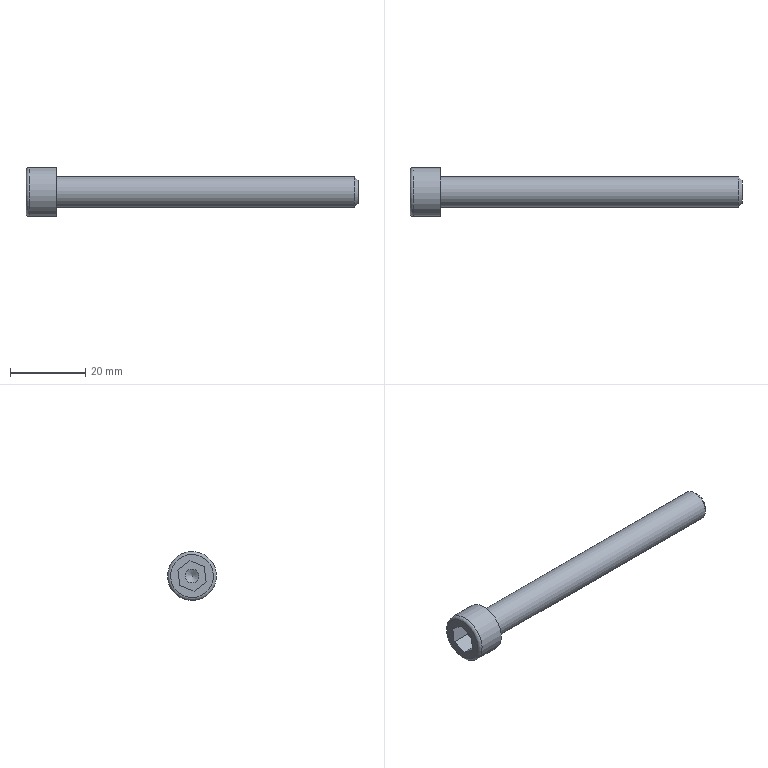Component | NX | GB_T70_1_M8X80_3 | 1 solid | 15 faces | box 88 x 13 x 13 mm | volume 4850 mm3 | plane 10 | cylinder 2 | cone 2 | torus 1 | commonest cylinder face diameters 13 x1 8 x1
STEP:
#1=CARTESIAN_POINT('',(0.,0.,0.));
#2=DIRECTION('',(0.,0.,1.));
#3=DIRECTION('',(1.,0.,0.));
#4=AXIS2_PLACEMENT_3D('',#1,#2,#3);
#5=CARTESIAN_POINT('',(-13.,24.732,-12.177));
#6=VERTEX_POINT('',#5);
#7=CARTESIAN_POINT('',(-13.,30.,-10.));
#8=DIRECTION('',(-1.,0.,0.));
#9=DIRECTION('',(0.,-0.9242,-0.3818));
#10=AXIS2_PLACEMENT_3D('',#7,#8,#9);
#11=CIRCLE('',#10,5.7);
#12=CARTESIAN_POINT('',(-13.,30.,-10.));
#13=DIRECTION('',(1.,0.,0.));
#14=DIRECTION('',(0.,-0.9242,-0.3818));
#15=AXIS2_PLACEMENT_3D('',#12,#13,#14);
#16=PLANE('',#15);
#17=CARTESIAN_POINT('',(5.7,0.));
#18=CARTESIAN_POINT('',(5.7,-9.873));
#19=CARTESIAN_POINT('',(-2.85,-4.936));
#20=CARTESIAN_POINT('',(-11.4,-0.));
#21=CARTESIAN_POINT('',(-2.85,4.936));
#22=CARTESIAN_POINT('',(5.7,9.873));
#23=CARTESIAN_POINT('',(5.7,0.));
#24=(BOUNDED_CURVE()B_SPLINE_CURVE(2,(#17,#18,#19,#20,#21,#22,#23),.UNSPECIFIED.,.T.,.F.)B_SPLINE_CURVE_WITH_KNOTS((1,2,2,2,2,1),(-2.094,0.,2.094,4.189,6.283,8.378),.UNSPECIFIED.)CURVE()GEOMETRIC_REPRESENTATION_ITEM()RATIONAL_B_SPLINE_CURVE((1.,0.5,1.,0.5,1.,0.5,1.))REPRESENTATION_ITEM(''));
#25=(GEOMETRIC_REPRESENTATION_CONTEXT(2)PARAMETRIC_REPRESENTATION_CONTEXT()REPRESENTATION_CONTEXT('',''));
#26=DEFINITIONAL_REPRESENTATION('',(#24),#25);
#27=PCURVE('',#16,#26);
#28=CARTESIAN_POINT('',(-12.2,30.,-10.));
#29=DIRECTION('',(1.,0.,0.));
#30=DIRECTION('',(0.,-0.9242,-0.3818));
#31=AXIS2_PLACEMENT_3D('',#28,#29,#30);
#32=TOROIDAL_SURFACE('',#31,5.7,0.8);
#33=CARTESIAN_POINT('',(6.283,4.712));
#34=DIRECTION('',(-1.,0.));
#35=VECTOR('',#34,1.);
#36=LINE('',#33,#35);
#37=(GEOMETRIC_REPRESENTATION_CONTEXT(2)PARAMETRIC_REPRESENTATION_CONTEXT()REPRESENTATION_CONTEXT('',''));
#38=DEFINITIONAL_REPRESENTATION('',(#36),#37);
#39=PCURVE('',#32,#38);
#40=SURFACE_CURVE('',#11,(#27,#39),.PCURVE_S1.);
#41=EDGE_CURVE('',#6,#6,#40,.T.);
#42=ORIENTED_EDGE('',*,*,#41,.T.);
#43=EDGE_LOOP('',(#42));
#44=FACE_BOUND('',#43,.T.);
#45=CARTESIAN_POINT('',(-13.,26.265,-11.543));
#46=VERTEX_POINT('',#45);
#47=CARTESIAN_POINT('',(-13.,26.796,-7.537));
#48=VERTEX_POINT('',#47);
#49=CARTESIAN_POINT('',(-13.,26.265,-11.543));
#50=DIRECTION('',(0.,0.1314,0.9913));
#51=VECTOR('',#50,1.);
#52=LINE('',#49,#51);
#53=CARTESIAN_POINT('',(4.041,0.));
#54=DIRECTION('',(-0.5,-0.866));
#55=VECTOR('',#54,1.);
#56=LINE('',#53,#55);
#57=(GEOMETRIC_REPRESENTATION_CONTEXT(2)PARAMETRIC_REPRESENTATION_CONTEXT()REPRESENTATION_CONTEXT('',''));
#58=DEFINITIONAL_REPRESENTATION('',(#56),#57);
#59=PCURVE('',#16,#58);
#60=CARTESIAN_POINT('',(-8.,26.265,-11.543));
#61=DIRECTION('',(0.,-0.9913,0.1314));
#62=DIRECTION('',(0.,0.1314,0.9913));
#63=AXIS2_PLACEMENT_3D('',#60,#61,#62);
#64=PLANE('',#63);
#65=CARTESIAN_POINT('',(0.,5.));
#66=DIRECTION('',(1.,0.));
#67=VECTOR('',#66,1.);
#68=LINE('',#65,#67);
#69=(GEOMETRIC_REPRESENTATION_CONTEXT(2)PARAMETRIC_REPRESENTATION_CONTEXT()REPRESENTATION_CONTEXT('',''));
#70=DEFINITIONAL_REPRESENTATION('',(#68),#69);
#71=PCURVE('',#64,#70);
#72=SURFACE_CURVE('',#52,(#59,#71),.PCURVE_S1.);
#73=EDGE_CURVE('',#46,#48,#72,.T.);
#74=ORIENTED_EDGE('',*,*,#73,.F.);
#75=CARTESIAN_POINT('',(-13.,29.469,-14.006));
#76=VERTEX_POINT('',#75);
#77=CARTESIAN_POINT('',(-13.,29.469,-14.006));
#78=DIRECTION('',(0.,-0.7928,0.6095));
#79=VECTOR('',#78,1.);
#80=LINE('',#77,#79);
#81=CARTESIAN_POINT('',(2.021,3.5));
#82=DIRECTION('',(0.5,-0.866));
#83=VECTOR('',#82,1.);
#84=LINE('',#81,#83);
#85=(GEOMETRIC_REPRESENTATION_CONTEXT(2)PARAMETRIC_REPRESENTATION_CONTEXT()REPRESENTATION_CONTEXT('',''));
#86=DEFINITIONAL_REPRESENTATION('',(#84),#85);
#87=PCURVE('',#16,#86);
#88=CARTESIAN_POINT('',(-8.,29.469,-14.006));
#89=DIRECTION('',(0.,-0.6095,-0.7928));
#90=DIRECTION('',(0.,-0.7928,0.6095));
#91=AXIS2_PLACEMENT_3D('',#88,#89,#90);
#92=PLANE('',#91);
#93=CARTESIAN_POINT('',(0.,5.));
#94=DIRECTION('',(1.,0.));
#95=VECTOR('',#94,1.);
#96=LINE('',#93,#95);
#97=(GEOMETRIC_REPRESENTATION_CONTEXT(2)PARAMETRIC_REPRESENTATION_CONTEXT()REPRESENTATION_CONTEXT('',''));
#98=DEFINITIONAL_REPRESENTATION('',(#96),#97);
#99=PCURVE('',#92,#98);
#100=SURFACE_CURVE('',#80,(#87,#99),.PCURVE_S1.);
#101=EDGE_CURVE('',#76,#46,#100,.T.);
#102=ORIENTED_EDGE('',*,*,#101,.F.);
#103=CARTESIAN_POINT('',(-13.,33.204,-12.463));
#104=VERTEX_POINT('',#103);
#105=CARTESIAN_POINT('',(-13.,33.204,-12.463));
#106=DIRECTION('',(0.,-0.9242,-0.3818));
#107=VECTOR('',#106,1.);
#108=LINE('',#105,#107);
#109=CARTESIAN_POINT('',(-2.021,3.5));
#110=DIRECTION('',(1.,0.));
#111=VECTOR('',#110,1.);
#112=LINE('',#109,#111);
#113=(GEOMETRIC_REPRESENTATION_CONTEXT(2)PARAMETRIC_REPRESENTATION_CONTEXT()REPRESENTATION_CONTEXT('',''));
#114=DEFINITIONAL_REPRESENTATION('',(#112),#113);
#115=PCURVE('',#16,#114);
#116=CARTESIAN_POINT('',(-8.,33.204,-12.463));
#117=DIRECTION('',(0.,0.3818,-0.9242));
#118=DIRECTION('',(0.,-0.9242,-0.3818));
#119=AXIS2_PLACEMENT_3D('',#116,#117,#118);
#120=PLANE('',#119);
#121=CARTESIAN_POINT('',(0.,5.));
#122=DIRECTION('',(1.,0.));
#123=VECTOR('',#122,1.);
#124=LINE('',#121,#123);
#125=(GEOMETRIC_REPRESENTATION_CONTEXT(2)PARAMETRIC_REPRESENTATION_CONTEXT()REPRESENTATION_CONTEXT('',''));
#126=DEFINITIONAL_REPRESENTATION('',(#124),#125);
#127=PCURVE('',#120,#126);
#128=SURFACE_CURVE('',#108,(#115,#127),.PCURVE_S1.);
#129=EDGE_CURVE('',#104,#76,#128,.T.);
#130=ORIENTED_EDGE('',*,*,#129,.F.);
#131=CARTESIAN_POINT('',(-13.,33.735,-8.457));
#132=VERTEX_POINT('',#131);
#133=CARTESIAN_POINT('',(-13.,33.735,-8.457));
#134=DIRECTION('',(0.,-0.1314,-0.9913));
#135=VECTOR('',#134,1.);
#136=LINE('',#133,#135);
#137=CARTESIAN_POINT('',(-4.041,-0.));
#138=DIRECTION('',(0.5,0.866));
#139=VECTOR('',#138,1.);
#140=LINE('',#137,#139);
#141=(GEOMETRIC_REPRESENTATION_CONTEXT(2)PARAMETRIC_REPRESENTATION_CONTEXT()REPRESENTATION_CONTEXT('',''));
#142=DEFINITIONAL_REPRESENTATION('',(#140),#141);
#143=PCURVE('',#16,#142);
#144=CARTESIAN_POINT('',(-8.,33.735,-8.457));
#145=DIRECTION('',(0.,0.9913,-0.1314));
#146=DIRECTION('',(0.,-0.1314,-0.9913));
#147=AXIS2_PLACEMENT_3D('',#144,#145,#146);
#148=PLANE('',#147);
#149=CARTESIAN_POINT('',(0.,5.));
#150=DIRECTION('',(1.,0.));
#151=VECTOR('',#150,1.);
#152=LINE('',#149,#151);
#153=(GEOMETRIC_REPRESENTATION_CONTEXT(2)PARAMETRIC_REPRESENTATION_CONTEXT()REPRESENTATION_CONTEXT('',''));
#154=DEFINITIONAL_REPRESENTATION('',(#152),#153);
#155=PCURVE('',#148,#154);
#156=SURFACE_CURVE('',#136,(#143,#155),.PCURVE_S1.);
#157=EDGE_CURVE('',#132,#104,#156,.T.);
#158=ORIENTED_EDGE('',*,*,#157,.F.);
#159=CARTESIAN_POINT('',(-13.,30.531,-5.994));
#160=VERTEX_POINT('',#159);
#161=CARTESIAN_POINT('',(-13.,30.531,-5.994));
#162=DIRECTION('',(0.,0.7928,-0.6095));
#163=VECTOR('',#162,1.);
#164=LINE('',#161,#163);
#165=CARTESIAN_POINT('',(-2.021,-3.5));
#166=DIRECTION('',(-0.5,0.866));
#167=VECTOR('',#166,1.);
#168=LINE('',#165,#167);
#169=(GEOMETRIC_REPRESENTATION_CONTEXT(2)PARAMETRIC_REPRESENTATION_CONTEXT()REPRESENTATION_CONTEXT('',''));
#170=DEFINITIONAL_REPRESENTATION('',(#168),#169);
#171=PCURVE('',#16,#170);
#172=CARTESIAN_POINT('',(-8.,30.531,-5.994));
#173=DIRECTION('',(0.,0.6095,0.7928));
#174=DIRECTION('',(0.,0.7928,-0.6095));
#175=AXIS2_PLACEMENT_3D('',#172,#173,#174);
#176=PLANE('',#175);
#177=CARTESIAN_POINT('',(0.,5.));
#178=DIRECTION('',(1.,0.));
#179=VECTOR('',#178,1.);
#180=LINE('',#177,#179);
#181=(GEOMETRIC_REPRESENTATION_CONTEXT(2)PARAMETRIC_REPRESENTATION_CONTEXT()REPRESENTATION_CONTEXT('',''));
#182=DEFINITIONAL_REPRESENTATION('',(#180),#181);
#183=PCURVE('',#176,#182);
#184=SURFACE_CURVE('',#164,(#171,#183),.PCURVE_S1.);
#185=EDGE_CURVE('',#160,#132,#184,.T.);
#186=ORIENTED_EDGE('',*,*,#185,.F.);
#187=CARTESIAN_POINT('',(-13.,26.796,-7.537));
#188=DIRECTION('',(0.,0.9242,0.3818));
#189=VECTOR('',#188,1.);
#190=LINE('',#187,#189);
#191=CARTESIAN_POINT('',(2.021,-3.5));
#192=DIRECTION('',(-1.,-0.));
#193=VECTOR('',#192,1.);
#194=LINE('',#191,#193);
#195=(GEOMETRIC_REPRESENTATION_CONTEXT(2)PARAMETRIC_REPRESENTATION_CONTEXT()REPRESENTATION_CONTEXT('',''));
#196=DEFINITIONAL_REPRESENTATION('',(#194),#195);
#197=PCURVE('',#16,#196);
#198=CARTESIAN_POINT('',(-8.,26.796,-7.537));
#199=DIRECTION('',(0.,-0.3818,0.9242));
#200=DIRECTION('',(0.,0.9242,0.3818));
#201=AXIS2_PLACEMENT_3D('',#198,#199,#200);
#202=PLANE('',#201);
#203=CARTESIAN_POINT('',(0.,5.));
#204=DIRECTION('',(1.,0.));
#205=VECTOR('',#204,1.);
#206=LINE('',#203,#205);
#207=(GEOMETRIC_REPRESENTATION_CONTEXT(2)PARAMETRIC_REPRESENTATION_CONTEXT()REPRESENTATION_CONTEXT('',''));
#208=DEFINITIONAL_REPRESENTATION('',(#206),#207);
#209=PCURVE('',#202,#208);
#210=SURFACE_CURVE('',#190,(#197,#209),.PCURVE_S1.);
#211=EDGE_CURVE('',#48,#160,#210,.T.);
#212=ORIENTED_EDGE('',*,*,#211,.F.);
#213=EDGE_LOOP('',(#74,#102,#130,#158,#186,#212));
#214=FACE_BOUND('',#213,.T.);
#215=ADVANCED_FACE('',(#44,#214),#16,.F.);
#216=CARTESIAN_POINT('',(-12.2,23.993,-12.482));
#217=VERTEX_POINT('',#216);
#218=CARTESIAN_POINT('',(-12.2,30.,-10.));
#219=DIRECTION('',(1.,0.,0.));
#220=DIRECTION('',(0.,-0.9242,-0.3818));
#221=AXIS2_PLACEMENT_3D('',#218,#219,#220);
#222=CIRCLE('',#221,6.5);
#223=CARTESIAN_POINT('',(75.,30.,-10.));
#224=DIRECTION('',(1.,0.,0.));
#225=DIRECTION('',(0.,-0.9242,-0.3818));
#226=AXIS2_PLACEMENT_3D('',#223,#224,#225);
#227=CYLINDRICAL_SURFACE('',#226,6.5);
#228=CARTESIAN_POINT('',(0.,-87.2));
#229=DIRECTION('',(1.,0.));
#230=VECTOR('',#229,1.);
#231=LINE('',#228,#230);
#232=(GEOMETRIC_REPRESENTATION_CONTEXT(2)PARAMETRIC_REPRESENTATION_CONTEXT()REPRESENTATION_CONTEXT('',''));
#233=DEFINITIONAL_REPRESENTATION('',(#231),#232);
#234=PCURVE('',#227,#233);
#235=CARTESIAN_POINT('',(0.,6.283));
#236=DIRECTION('',(1.,0.));
#237=VECTOR('',#236,1.);
#238=LINE('',#235,#237);
#239=(GEOMETRIC_REPRESENTATION_CONTEXT(2)PARAMETRIC_REPRESENTATION_CONTEXT()REPRESENTATION_CONTEXT('',''));
#240=DEFINITIONAL_REPRESENTATION('',(#238),#239);
#241=PCURVE('',#32,#240);
#242=SURFACE_CURVE('',#222,(#234,#241),.PCURVE_S1.);
#243=EDGE_CURVE('',#217,#217,#242,.T.);
#244=ORIENTED_EDGE('',*,*,#243,.T.);
#245=CARTESIAN_POINT('',(-5.,23.993,-12.482));
#246=VERTEX_POINT('',#245);
#247=CARTESIAN_POINT('',(-12.2,23.993,-12.482));
#248=CARTESIAN_POINT('',(-5.,23.993,-12.482));
#249=B_SPLINE_CURVE_WITH_KNOTS('',1,(#247,#248),.UNSPECIFIED.,.F.,.F.,(2,2),(-87.2,-80.),.PIECEWISE_BEZIER_KNOTS.);
#250=CARTESIAN_POINT('',(6.283,0.));
#251=DIRECTION('',(0.,1.));
#252=VECTOR('',#251,1.);
#253=LINE('',#250,#252);
#254=(GEOMETRIC_REPRESENTATION_CONTEXT(2)PARAMETRIC_REPRESENTATION_CONTEXT()REPRESENTATION_CONTEXT('',''));
#255=DEFINITIONAL_REPRESENTATION('',(#253),#254);
#256=PCURVE('',#227,#255);
#257=CARTESIAN_POINT('',(0.,0.));
#258=DIRECTION('',(0.,1.));
#259=VECTOR('',#258,1.);
#260=LINE('',#257,#259);
#261=(GEOMETRIC_REPRESENTATION_CONTEXT(2)PARAMETRIC_REPRESENTATION_CONTEXT()REPRESENTATION_CONTEXT('',''));
#262=DEFINITIONAL_REPRESENTATION('',(#260),#261);
#263=PCURVE('',#227,#262);
#264=SEAM_CURVE('',#249,(#256,#263),.PCURVE_S1.);
#265=EDGE_CURVE('',#217,#246,#264,.T.);
#266=ORIENTED_EDGE('',*,*,#265,.T.);
#267=CARTESIAN_POINT('',(-5.,30.,-10.));
#268=DIRECTION('',(1.,0.,0.));
#269=DIRECTION('',(0.,-0.9242,-0.3818));
#270=AXIS2_PLACEMENT_3D('',#267,#268,#269);
#271=CIRCLE('',#270,6.5);
#272=CARTESIAN_POINT('',(0.,-80.));
#273=DIRECTION('',(1.,0.));
#274=VECTOR('',#273,1.);
#275=LINE('',#272,#274);
#276=(GEOMETRIC_REPRESENTATION_CONTEXT(2)PARAMETRIC_REPRESENTATION_CONTEXT()REPRESENTATION_CONTEXT('',''));
#277=DEFINITIONAL_REPRESENTATION('',(#275),#276);
#278=PCURVE('',#227,#277);
#279=CARTESIAN_POINT('',(-5.,27.518,-3.993));
#280=DIRECTION('',(-1.,0.,0.));
#281=DIRECTION('',(0.,0.9242,0.3818));
#282=AXIS2_PLACEMENT_3D('',#279,#280,#281);
#283=PLANE('',#282);
#284=CARTESIAN_POINT('',(-6.5,6.5));
#285=CARTESIAN_POINT('',(-6.5,17.758));
#286=CARTESIAN_POINT('',(3.25,12.129));
#287=CARTESIAN_POINT('',(13.,6.5));
#288=CARTESIAN_POINT('',(3.25,0.8708));
#289=CARTESIAN_POINT('',(-6.5,-4.758));
#290=CARTESIAN_POINT('',(-6.5,6.5));
#291=(BOUNDED_CURVE()B_SPLINE_CURVE(2,(#284,#285,#286,#287,#288,#289,#290),.UNSPECIFIED.,.T.,.F.)B_SPLINE_CURVE_WITH_KNOTS((1,2,2,2,2,1),(-2.094,0.,2.094,4.189,6.283,8.378),.UNSPECIFIED.)CURVE()GEOMETRIC_REPRESENTATION_ITEM()RATIONAL_B_SPLINE_CURVE((1.,0.5,1.,0.5,1.,0.5,1.))REPRESENTATION_ITEM(''));
#292=(GEOMETRIC_REPRESENTATION_CONTEXT(2)PARAMETRIC_REPRESENTATION_CONTEXT()REPRESENTATION_CONTEXT('',''));
#293=DEFINITIONAL_REPRESENTATION('',(#291),#292);
#294=PCURVE('',#283,#293);
#295=SURFACE_CURVE('',#271,(#278,#294),.PCURVE_S1.);
#296=EDGE_CURVE('',#246,#246,#295,.T.);
#297=ORIENTED_EDGE('',*,*,#296,.F.);
#298=ORIENTED_EDGE('',*,*,#265,.F.);
#299=EDGE_LOOP('',(#244,#266,#297,#298));
#300=FACE_BOUND('',#299,.T.);
#301=ADVANCED_FACE('',(#300),#227,.T.);
#302=CARTESIAN_POINT('',(-5.,26.303,-11.527));
#303=VERTEX_POINT('',#302);
#304=CARTESIAN_POINT('',(-5.,30.,-10.));
#305=DIRECTION('',(1.,0.,0.));
#306=DIRECTION('',(0.,-0.9242,-0.3818));
#307=AXIS2_PLACEMENT_3D('',#304,#305,#306);
#308=CIRCLE('',#307,4.);
#309=CARTESIAN_POINT('',(-4.,6.5));
#310=CARTESIAN_POINT('',(-4.,13.428));
#311=CARTESIAN_POINT('',(2.,9.964));
#312=CARTESIAN_POINT('',(8.,6.5));
#313=CARTESIAN_POINT('',(2.,3.036));
#314=CARTESIAN_POINT('',(-4.,-0.4282));
#315=CARTESIAN_POINT('',(-4.,6.5));
#316=(BOUNDED_CURVE()B_SPLINE_CURVE(2,(#309,#310,#311,#312,#313,#314,#315),.UNSPECIFIED.,.T.,.F.)B_SPLINE_CURVE_WITH_KNOTS((1,2,2,2,2,1),(-2.094,0.,2.094,4.189,6.283,8.378),.UNSPECIFIED.)CURVE()GEOMETRIC_REPRESENTATION_ITEM()RATIONAL_B_SPLINE_CURVE((1.,0.5,1.,0.5,1.,0.5,1.))REPRESENTATION_ITEM(''));
#317=(GEOMETRIC_REPRESENTATION_CONTEXT(2)PARAMETRIC_REPRESENTATION_CONTEXT()REPRESENTATION_CONTEXT('',''));
#318=DEFINITIONAL_REPRESENTATION('',(#316),#317);
#319=PCURVE('',#283,#318);
#320=CARTESIAN_POINT('',(75.,30.,-10.));
#321=DIRECTION('',(1.,0.,0.));
#322=DIRECTION('',(0.,-0.9242,-0.3818));
#323=AXIS2_PLACEMENT_3D('',#320,#321,#322);
#324=CYLINDRICAL_SURFACE('',#323,4.);
#325=CARTESIAN_POINT('',(0.,-80.));
#326=DIRECTION('',(1.,0.));
#327=VECTOR('',#326,1.);
#328=LINE('',#325,#327);
#329=(GEOMETRIC_REPRESENTATION_CONTEXT(2)PARAMETRIC_REPRESENTATION_CONTEXT()REPRESENTATION_CONTEXT('',''));
#330=DEFINITIONAL_REPRESENTATION('',(#328),#329);
#331=PCURVE('',#324,#330);
#332=SURFACE_CURVE('',#308,(#319,#331),.PCURVE_S1.);
#333=EDGE_CURVE('',#303,#303,#332,.T.);
#334=ORIENTED_EDGE('',*,*,#333,.F.);
#335=EDGE_LOOP('',(#334));
#336=FACE_BOUND('',#335,.T.);
#337=ORIENTED_EDGE('',*,*,#296,.T.);
#338=EDGE_LOOP('',(#337));
#339=FACE_BOUND('',#338,.T.);
#340=ADVANCED_FACE('',(#336,#339),#283,.F.);
#341=CARTESIAN_POINT('',(74.,33.697,-8.473));
#342=VERTEX_POINT('',#341);
#343=CARTESIAN_POINT('',(74.,26.303,-11.527));
#344=VERTEX_POINT('',#343);
#345=CARTESIAN_POINT('',(74.,30.,-10.));
#346=DIRECTION('',(-1.,0.,0.));
#347=DIRECTION('',(0.,0.9242,0.3818));
#348=AXIS2_PLACEMENT_3D('',#345,#346,#347);
#349=CIRCLE('',#348,4.);
#350=CARTESIAN_POINT('',(3.142,-1.));
#351=DIRECTION('',(-1.,0.));
#352=VECTOR('',#351,1.);
#353=LINE('',#350,#352);
#354=(GEOMETRIC_REPRESENTATION_CONTEXT(2)PARAMETRIC_REPRESENTATION_CONTEXT()REPRESENTATION_CONTEXT('',''));
#355=DEFINITIONAL_REPRESENTATION('',(#353),#354);
#356=PCURVE('',#324,#355);
#357=CARTESIAN_POINT('',(75.,30.,-10.));
#358=DIRECTION('',(-1.,0.,0.));
#359=DIRECTION('',(0.,0.9242,0.3818));
#360=AXIS2_PLACEMENT_3D('',#357,#358,#359);
#361=CONICAL_SURFACE('',#360,3.,0.7854);
#362=CARTESIAN_POINT('',(0.,1.));
#363=DIRECTION('',(1.,0.));
#364=VECTOR('',#363,1.);
#365=LINE('',#362,#364);
#366=(GEOMETRIC_REPRESENTATION_CONTEXT(2)PARAMETRIC_REPRESENTATION_CONTEXT()REPRESENTATION_CONTEXT('',''));
#367=DEFINITIONAL_REPRESENTATION('',(#365),#366);
#368=PCURVE('',#361,#367);
#369=SURFACE_CURVE('',#349,(#356,#368),.PCURVE_S1.);
#370=EDGE_CURVE('',#342,#344,#369,.T.);
#371=ORIENTED_EDGE('',*,*,#370,.T.);
#372=CARTESIAN_POINT('',(-5.,26.303,-11.527));
#373=CARTESIAN_POINT('',(74.,26.303,-11.527));
#374=B_SPLINE_CURVE_WITH_KNOTS('',1,(#372,#373),.UNSPECIFIED.,.F.,.F.,(2,2),(-80.,-1.),.PIECEWISE_BEZIER_KNOTS.);
#375=CARTESIAN_POINT('',(0.,0.));
#376=DIRECTION('',(0.,1.));
#377=VECTOR('',#376,1.);
#378=LINE('',#375,#377);
#379=(GEOMETRIC_REPRESENTATION_CONTEXT(2)PARAMETRIC_REPRESENTATION_CONTEXT()REPRESENTATION_CONTEXT('',''));
#380=DEFINITIONAL_REPRESENTATION('',(#378),#379);
#381=PCURVE('',#324,#380);
#382=CARTESIAN_POINT('',(6.283,0.));
#383=DIRECTION('',(0.,1.));
#384=VECTOR('',#383,1.);
#385=LINE('',#382,#384);
#386=(GEOMETRIC_REPRESENTATION_CONTEXT(2)PARAMETRIC_REPRESENTATION_CONTEXT()REPRESENTATION_CONTEXT('',''));
#387=DEFINITIONAL_REPRESENTATION('',(#385),#386);
#388=PCURVE('',#324,#387);
#389=SEAM_CURVE('',#374,(#381,#388),.PCURVE_S1.);
#390=EDGE_CURVE('',#303,#344,#389,.T.);
#391=ORIENTED_EDGE('',*,*,#390,.F.);
#392=ORIENTED_EDGE('',*,*,#333,.T.);
#393=ORIENTED_EDGE('',*,*,#390,.T.);
#394=CARTESIAN_POINT('',(74.,30.,-10.));
#395=DIRECTION('',(-1.,0.,0.));
#396=DIRECTION('',(0.,0.9242,0.3818));
#397=AXIS2_PLACEMENT_3D('',#394,#395,#396);
#398=CIRCLE('',#397,4.);
#399=CARTESIAN_POINT('',(9.425,-1.));
#400=DIRECTION('',(-1.,0.));
#401=VECTOR('',#400,1.);
#402=LINE('',#399,#401);
#403=(GEOMETRIC_REPRESENTATION_CONTEXT(2)PARAMETRIC_REPRESENTATION_CONTEXT()REPRESENTATION_CONTEXT('',''));
#404=DEFINITIONAL_REPRESENTATION('',(#402),#403);
#405=PCURVE('',#324,#404);
#406=CARTESIAN_POINT('',(0.,1.));
#407=DIRECTION('',(1.,0.));
#408=VECTOR('',#407,1.);
#409=LINE('',#406,#408);
#410=(GEOMETRIC_REPRESENTATION_CONTEXT(2)PARAMETRIC_REPRESENTATION_CONTEXT()REPRESENTATION_CONTEXT('',''));
#411=DEFINITIONAL_REPRESENTATION('',(#409),#410);
#412=PCURVE('',#361,#411);
#413=SURFACE_CURVE('',#398,(#405,#412),.PCURVE_S1.);
#414=EDGE_CURVE('',#344,#342,#413,.T.);
#415=ORIENTED_EDGE('',*,*,#414,.T.);
#416=EDGE_LOOP('',(#371,#391,#392,#393,#415));
#417=FACE_BOUND('',#416,.T.);
#418=ADVANCED_FACE('',(#417),#324,.T.);
#419=CARTESIAN_POINT('',(75.,32.773,-8.854));
#420=VERTEX_POINT('',#419);
#421=CARTESIAN_POINT('',(75.,30.,-10.));
#422=DIRECTION('',(1.,0.,0.));
#423=DIRECTION('',(0.,0.9242,0.3818));
#424=AXIS2_PLACEMENT_3D('',#421,#422,#423);
#425=CIRCLE('',#424,3.);
#426=CARTESIAN_POINT('',(75.,28.473,-6.303));
#427=DIRECTION('',(-1.,0.,0.));
#428=DIRECTION('',(0.,0.9242,0.3818));
#429=AXIS2_PLACEMENT_3D('',#426,#427,#428);
#430=PLANE('',#429);
#431=CARTESIAN_POINT('',(3.,4.));
#432=CARTESIAN_POINT('',(3.,-1.196));
#433=CARTESIAN_POINT('',(-1.5,1.402));
#434=CARTESIAN_POINT('',(-6.,4.));
#435=CARTESIAN_POINT('',(-1.5,6.598));
#436=CARTESIAN_POINT('',(3.,9.196));
#437=CARTESIAN_POINT('',(3.,4.));
#438=(BOUNDED_CURVE()B_SPLINE_CURVE(2,(#431,#432,#433,#434,#435,#436,#437),.UNSPECIFIED.,.T.,.F.)B_SPLINE_CURVE_WITH_KNOTS((1,2,2,2,2,1),(-2.094,0.,2.094,4.189,6.283,8.378),.UNSPECIFIED.)CURVE()GEOMETRIC_REPRESENTATION_ITEM()RATIONAL_B_SPLINE_CURVE((1.,0.5,1.,0.5,1.,0.5,1.))REPRESENTATION_ITEM(''));
#439=(GEOMETRIC_REPRESENTATION_CONTEXT(2)PARAMETRIC_REPRESENTATION_CONTEXT()REPRESENTATION_CONTEXT('',''));
#440=DEFINITIONAL_REPRESENTATION('',(#438),#439);
#441=PCURVE('',#430,#440);
#442=CARTESIAN_POINT('',(6.283,0.));
#443=DIRECTION('',(-1.,-0.));
#444=VECTOR('',#443,1.);
#445=LINE('',#442,#444);
#446=(GEOMETRIC_REPRESENTATION_CONTEXT(2)PARAMETRIC_REPRESENTATION_CONTEXT()REPRESENTATION_CONTEXT('',''));
#447=DEFINITIONAL_REPRESENTATION('',(#445),#446);
#448=PCURVE('',#361,#447);
#449=SURFACE_CURVE('',#425,(#441,#448),.PCURVE_S1.);
#450=EDGE_CURVE('',#420,#420,#449,.T.);
#451=ORIENTED_EDGE('',*,*,#450,.T.);
#452=EDGE_LOOP('',(#451));
#453=FACE_BOUND('',#452,.T.);
#454=ADVANCED_FACE('',(#453),#430,.F.);
#455=ORIENTED_EDGE('',*,*,#41,.F.);
#456=CARTESIAN_POINT('',(-13.,24.732,-12.177));
#457=CARTESIAN_POINT('',(-13.,24.534,-12.258));
#458=CARTESIAN_POINT('',(-12.932,24.342,-12.338));
#459=CARTESIAN_POINT('',(-12.802,24.176,-12.406));
#460=CARTESIAN_POINT('',(-12.622,24.055,-12.456));
#461=CARTESIAN_POINT('',(-12.414,23.993,-12.482));
#462=CARTESIAN_POINT('',(-12.2,23.993,-12.482));
#463=(BOUNDED_CURVE()B_SPLINE_CURVE(6,(#456,#457,#458,#459,#460,#461,#462),.UNSPECIFIED.,.F.,.F.)B_SPLINE_CURVE_WITH_KNOTS((7,7),(4.712,6.283),.PIECEWISE_BEZIER_KNOTS.)CURVE()GEOMETRIC_REPRESENTATION_ITEM()RATIONAL_B_SPLINE_CURVE((1.031,1.01,0.9979,0.994,0.9979,1.01,1.031))REPRESENTATION_ITEM(''));
#464=CARTESIAN_POINT('',(6.283,0.));
#465=DIRECTION('',(0.,1.));
#466=VECTOR('',#465,1.);
#467=LINE('',#464,#466);
#468=(GEOMETRIC_REPRESENTATION_CONTEXT(2)PARAMETRIC_REPRESENTATION_CONTEXT()REPRESENTATION_CONTEXT('',''));
#469=DEFINITIONAL_REPRESENTATION('',(#467),#468);
#470=PCURVE('',#32,#469);
#471=CARTESIAN_POINT('',(0.,0.));
#472=DIRECTION('',(0.,1.));
#473=VECTOR('',#472,1.);
#474=LINE('',#471,#473);
#475=(GEOMETRIC_REPRESENTATION_CONTEXT(2)PARAMETRIC_REPRESENTATION_CONTEXT()REPRESENTATION_CONTEXT('',''));
#476=DEFINITIONAL_REPRESENTATION('',(#474),#475);
#477=PCURVE('',#32,#476);
#478=SEAM_CURVE('',#463,(#470,#477),.PCURVE_S1.);
#479=EDGE_CURVE('',#6,#217,#478,.T.);
#480=ORIENTED_EDGE('',*,*,#479,.T.);
#481=ORIENTED_EDGE('',*,*,#243,.F.);
#482=ORIENTED_EDGE('',*,*,#479,.F.);
#483=EDGE_LOOP('',(#455,#480,#481,#482));
#484=FACE_BOUND('',#483,.T.);
#485=ADVANCED_FACE('',(#484),#32,.T.);
#486=ORIENTED_EDGE('',*,*,#370,.F.);
#487=CARTESIAN_POINT('',(75.,32.773,-8.854));
#488=CARTESIAN_POINT('',(74.,33.697,-8.473));
#489=B_SPLINE_CURVE_WITH_KNOTS('',1,(#487,#488),.UNSPECIFIED.,.F.,.F.,(2,2),(0.,1.414),.PIECEWISE_BEZIER_KNOTS.);
#490=CARTESIAN_POINT('',(0.,0.));
#491=DIRECTION('',(0.,1.));
#492=VECTOR('',#491,1.);
#493=LINE('',#490,#492);
#494=(GEOMETRIC_REPRESENTATION_CONTEXT(2)PARAMETRIC_REPRESENTATION_CONTEXT()REPRESENTATION_CONTEXT('',''));
#495=DEFINITIONAL_REPRESENTATION('',(#493),#494);
#496=PCURVE('',#361,#495);
#497=CARTESIAN_POINT('',(6.283,0.));
#498=DIRECTION('',(0.,1.));
#499=VECTOR('',#498,1.);
#500=LINE('',#497,#499);
#501=(GEOMETRIC_REPRESENTATION_CONTEXT(2)PARAMETRIC_REPRESENTATION_CONTEXT()REPRESENTATION_CONTEXT('',''));
#502=DEFINITIONAL_REPRESENTATION('',(#500),#501);
#503=PCURVE('',#361,#502);
#504=SEAM_CURVE('',#489,(#496,#503),.PCURVE_S1.);
#505=EDGE_CURVE('',#420,#342,#504,.T.);
#506=ORIENTED_EDGE('',*,*,#505,.F.);
#507=ORIENTED_EDGE('',*,*,#450,.F.);
#508=ORIENTED_EDGE('',*,*,#505,.T.);
#509=ORIENTED_EDGE('',*,*,#414,.F.);
#510=EDGE_LOOP('',(#486,#506,#507,#508,#509));
#511=FACE_BOUND('',#510,.T.);
#512=ADVANCED_FACE('',(#511),#361,.T.);
#513=CARTESIAN_POINT('',(-8.,26.796,-7.537));
#514=VERTEX_POINT('',#513);
#515=CARTESIAN_POINT('',(-8.,26.265,-11.543));
#516=VERTEX_POINT('',#515);
#517=CARTESIAN_POINT('',(-8.,26.265,-11.543));
#518=DIRECTION('',(0.,-0.1314,-0.9913));
#519=VECTOR('',#518,1.);
#520=LINE('',#517,#519);
#521=CARTESIAN_POINT('',(-8.,30.,-10.));
#522=DIRECTION('',(-1.,0.,0.));
#523=DIRECTION('',(0.,0.9242,0.3818));
#524=AXIS2_PLACEMENT_3D('',#521,#522,#523);
#525=PLANE('',#524);
#526=CARTESIAN_POINT('',(-4.041,0.));
#527=DIRECTION('',(-0.5,0.866));
#528=VECTOR('',#527,1.);
#529=LINE('',#526,#528);
#530=(GEOMETRIC_REPRESENTATION_CONTEXT(2)PARAMETRIC_REPRESENTATION_CONTEXT()REPRESENTATION_CONTEXT('',''));
#531=DEFINITIONAL_REPRESENTATION('',(#529),#530);
#532=PCURVE('',#525,#531);
#533=CARTESIAN_POINT('',(0.,0.));
#534=DIRECTION('',(-1.,0.));
#535=VECTOR('',#534,1.);
#536=LINE('',#533,#535);
#537=(GEOMETRIC_REPRESENTATION_CONTEXT(2)PARAMETRIC_REPRESENTATION_CONTEXT()REPRESENTATION_CONTEXT('',''));
#538=DEFINITIONAL_REPRESENTATION('',(#536),#537);
#539=PCURVE('',#64,#538);
#540=SURFACE_CURVE('',#520,(#532,#539),.PCURVE_S1.);
#541=EDGE_CURVE('',#514,#516,#540,.T.);
#542=ORIENTED_EDGE('',*,*,#541,.F.);
#543=CARTESIAN_POINT('',(-8.,30.531,-5.994));
#544=VERTEX_POINT('',#543);
#545=CARTESIAN_POINT('',(-8.,26.796,-7.537));
#546=DIRECTION('',(0.,-0.9242,-0.3818));
#547=VECTOR('',#546,1.);
#548=LINE('',#545,#547);
#549=CARTESIAN_POINT('',(-2.021,-3.5));
#550=DIRECTION('',(-1.,0.));
#551=VECTOR('',#550,1.);
#552=LINE('',#549,#551);
#553=(GEOMETRIC_REPRESENTATION_CONTEXT(2)PARAMETRIC_REPRESENTATION_CONTEXT()REPRESENTATION_CONTEXT('',''));
#554=DEFINITIONAL_REPRESENTATION('',(#552),#553);
#555=PCURVE('',#525,#554);
#556=CARTESIAN_POINT('',(0.,0.));
#557=DIRECTION('',(-1.,0.));
#558=VECTOR('',#557,1.);
#559=LINE('',#556,#558);
#560=(GEOMETRIC_REPRESENTATION_CONTEXT(2)PARAMETRIC_REPRESENTATION_CONTEXT()REPRESENTATION_CONTEXT('',''));
#561=DEFINITIONAL_REPRESENTATION('',(#559),#560);
#562=PCURVE('',#202,#561);
#563=SURFACE_CURVE('',#548,(#555,#562),.PCURVE_S1.);
#564=EDGE_CURVE('',#544,#514,#563,.T.);
#565=ORIENTED_EDGE('',*,*,#564,.F.);
#566=CARTESIAN_POINT('',(-8.,33.735,-8.457));
#567=VERTEX_POINT('',#566);
#568=CARTESIAN_POINT('',(-8.,30.531,-5.994));
#569=DIRECTION('',(0.,-0.7928,0.6095));
#570=VECTOR('',#569,1.);
#571=LINE('',#568,#570);
#572=CARTESIAN_POINT('',(2.021,-3.5));
#573=DIRECTION('',(-0.5,-0.866));
#574=VECTOR('',#573,1.);
#575=LINE('',#572,#574);
#576=(GEOMETRIC_REPRESENTATION_CONTEXT(2)PARAMETRIC_REPRESENTATION_CONTEXT()REPRESENTATION_CONTEXT('',''));
#577=DEFINITIONAL_REPRESENTATION('',(#575),#576);
#578=PCURVE('',#525,#577);
#579=CARTESIAN_POINT('',(0.,0.));
#580=DIRECTION('',(-1.,0.));
#581=VECTOR('',#580,1.);
#582=LINE('',#579,#581);
#583=(GEOMETRIC_REPRESENTATION_CONTEXT(2)PARAMETRIC_REPRESENTATION_CONTEXT()REPRESENTATION_CONTEXT('',''));
#584=DEFINITIONAL_REPRESENTATION('',(#582),#583);
#585=PCURVE('',#176,#584);
#586=SURFACE_CURVE('',#571,(#578,#585),.PCURVE_S1.);
#587=EDGE_CURVE('',#567,#544,#586,.T.);
#588=ORIENTED_EDGE('',*,*,#587,.F.);
#589=CARTESIAN_POINT('',(-8.,33.204,-12.463));
#590=VERTEX_POINT('',#589);
#591=CARTESIAN_POINT('',(-8.,33.735,-8.457));
#592=DIRECTION('',(0.,0.1314,0.9913));
#593=VECTOR('',#592,1.);
#594=LINE('',#591,#593);
#595=CARTESIAN_POINT('',(4.041,-0.));
#596=DIRECTION('',(0.5,-0.866));
#597=VECTOR('',#596,1.);
#598=LINE('',#595,#597);
#599=(GEOMETRIC_REPRESENTATION_CONTEXT(2)PARAMETRIC_REPRESENTATION_CONTEXT()REPRESENTATION_CONTEXT('',''));
#600=DEFINITIONAL_REPRESENTATION('',(#598),#599);
#601=PCURVE('',#525,#600);
#602=CARTESIAN_POINT('',(0.,0.));
#603=DIRECTION('',(-1.,0.));
#604=VECTOR('',#603,1.);
#605=LINE('',#602,#604);
#606=(GEOMETRIC_REPRESENTATION_CONTEXT(2)PARAMETRIC_REPRESENTATION_CONTEXT()REPRESENTATION_CONTEXT('',''));
#607=DEFINITIONAL_REPRESENTATION('',(#605),#606);
#608=PCURVE('',#148,#607);
#609=SURFACE_CURVE('',#594,(#601,#608),.PCURVE_S1.);
#610=EDGE_CURVE('',#590,#567,#609,.T.);
#611=ORIENTED_EDGE('',*,*,#610,.F.);
#612=CARTESIAN_POINT('',(-8.,29.469,-14.006));
#613=VERTEX_POINT('',#612);
#614=CARTESIAN_POINT('',(-8.,33.204,-12.463));
#615=DIRECTION('',(0.,0.9242,0.3818));
#616=VECTOR('',#615,1.);
#617=LINE('',#614,#616);
#618=CARTESIAN_POINT('',(2.021,3.5));
#619=DIRECTION('',(1.,-0.));
#620=VECTOR('',#619,1.);
#621=LINE('',#618,#620);
#622=(GEOMETRIC_REPRESENTATION_CONTEXT(2)PARAMETRIC_REPRESENTATION_CONTEXT()REPRESENTATION_CONTEXT('',''));
#623=DEFINITIONAL_REPRESENTATION('',(#621),#622);
#624=PCURVE('',#525,#623);
#625=CARTESIAN_POINT('',(0.,0.));
#626=DIRECTION('',(-1.,0.));
#627=VECTOR('',#626,1.);
#628=LINE('',#625,#627);
#629=(GEOMETRIC_REPRESENTATION_CONTEXT(2)PARAMETRIC_REPRESENTATION_CONTEXT()REPRESENTATION_CONTEXT('',''));
#630=DEFINITIONAL_REPRESENTATION('',(#628),#629);
#631=PCURVE('',#120,#630);
#632=SURFACE_CURVE('',#617,(#624,#631),.PCURVE_S1.);
#633=EDGE_CURVE('',#613,#590,#632,.T.);
#634=ORIENTED_EDGE('',*,*,#633,.F.);
#635=CARTESIAN_POINT('',(-8.,29.469,-14.006));
#636=DIRECTION('',(0.,0.7928,-0.6095));
#637=VECTOR('',#636,1.);
#638=LINE('',#635,#637);
#639=CARTESIAN_POINT('',(-2.021,3.5));
#640=DIRECTION('',(0.5,0.866));
#641=VECTOR('',#640,1.);
#642=LINE('',#639,#641);
#643=(GEOMETRIC_REPRESENTATION_CONTEXT(2)PARAMETRIC_REPRESENTATION_CONTEXT()REPRESENTATION_CONTEXT('',''));
#644=DEFINITIONAL_REPRESENTATION('',(#642),#643);
#645=PCURVE('',#525,#644);
#646=CARTESIAN_POINT('',(0.,0.));
#647=DIRECTION('',(-1.,0.));
#648=VECTOR('',#647,1.);
#649=LINE('',#646,#648);
#650=(GEOMETRIC_REPRESENTATION_CONTEXT(2)PARAMETRIC_REPRESENTATION_CONTEXT()REPRESENTATION_CONTEXT('',''));
#651=DEFINITIONAL_REPRESENTATION('',(#649),#650);
#652=PCURVE('',#92,#651);
#653=SURFACE_CURVE('',#638,(#645,#652),.PCURVE_S1.);
#654=EDGE_CURVE('',#516,#613,#653,.T.);
#655=ORIENTED_EDGE('',*,*,#654,.F.);
#656=EDGE_LOOP('',(#542,#565,#588,#611,#634,#655));
#657=FACE_BOUND('',#656,.T.);
#658=CARTESIAN_POINT('',(-8.,31.697,-9.299));
#659=VERTEX_POINT('',#658);
#660=CARTESIAN_POINT('',(-8.,30.,-10.));
#661=DIRECTION('',(-1.,0.,0.));
#662=DIRECTION('',(0.,0.9242,0.3818));
#663=AXIS2_PLACEMENT_3D('',#660,#661,#662);
#664=CIRCLE('',#663,1.836);
#665=CARTESIAN_POINT('',(0.,0.));
#666=DIRECTION('',(1.,0.));
#667=AXIS2_PLACEMENT_2D('',#665,#666);
#668=CIRCLE('',#667,1.836);
#669=(GEOMETRIC_REPRESENTATION_CONTEXT(2)PARAMETRIC_REPRESENTATION_CONTEXT()REPRESENTATION_CONTEXT('',''));
#670=DEFINITIONAL_REPRESENTATION('',(#668),#669);
#671=PCURVE('',#525,#670);
#672=CARTESIAN_POINT('',(-9.,30.,-10.));
#673=DIRECTION('',(-1.,0.,0.));
#674=DIRECTION('',(0.,0.9242,0.3818));
#675=AXIS2_PLACEMENT_3D('',#672,#673,#674);
#676=CONICAL_SURFACE('',#675,3.5,1.03);
#677=CARTESIAN_POINT('',(0.,-1.));
#678=DIRECTION('',(1.,0.));
#679=VECTOR('',#678,1.);
#680=LINE('',#677,#679);
#681=(GEOMETRIC_REPRESENTATION_CONTEXT(2)PARAMETRIC_REPRESENTATION_CONTEXT()REPRESENTATION_CONTEXT('',''));
#682=DEFINITIONAL_REPRESENTATION('',(#680),#681);
#683=PCURVE('',#676,#682);
#684=SURFACE_CURVE('',#664,(#671,#683),.PCURVE_S1.);
#685=EDGE_CURVE('',#659,#659,#684,.T.);
#686=ORIENTED_EDGE('',*,*,#685,.F.);
#687=EDGE_LOOP('',(#686));
#688=FACE_BOUND('',#687,.T.);
#689=ADVANCED_FACE('',(#657,#688),#525,.T.);
#690=CARTESIAN_POINT('',(-8.,26.265,-11.543));
#691=DIRECTION('',(1.,0.,0.));
#692=VECTOR('',#691,1.);
#693=LINE('',#690,#692);
#694=CARTESIAN_POINT('',(0.,0.));
#695=DIRECTION('',(0.,-1.));
#696=VECTOR('',#695,1.);
#697=LINE('',#694,#696);
#698=(GEOMETRIC_REPRESENTATION_CONTEXT(2)PARAMETRIC_REPRESENTATION_CONTEXT()REPRESENTATION_CONTEXT('',''));
#699=DEFINITIONAL_REPRESENTATION('',(#697),#698);
#700=PCURVE('',#64,#699);
#701=CARTESIAN_POINT('',(4.041,0.));
#702=DIRECTION('',(0.,-1.));
#703=VECTOR('',#702,1.);
#704=LINE('',#701,#703);
#705=(GEOMETRIC_REPRESENTATION_CONTEXT(2)PARAMETRIC_REPRESENTATION_CONTEXT()REPRESENTATION_CONTEXT('',''));
#706=DEFINITIONAL_REPRESENTATION('',(#704),#705);
#707=PCURVE('',#92,#706);
#708=SURFACE_CURVE('',#693,(#700,#707),.PCURVE_S1.);
#709=EDGE_CURVE('',#46,#516,#708,.T.);
#710=ORIENTED_EDGE('',*,*,#709,.F.);
#711=ORIENTED_EDGE('',*,*,#73,.T.);
#712=CARTESIAN_POINT('',(-8.,26.796,-7.537));
#713=DIRECTION('',(1.,0.,0.));
#714=VECTOR('',#713,1.);
#715=LINE('',#712,#714);
#716=CARTESIAN_POINT('',(4.041,0.));
#717=DIRECTION('',(0.,-1.));
#718=VECTOR('',#717,1.);
#719=LINE('',#716,#718);
#720=(GEOMETRIC_REPRESENTATION_CONTEXT(2)PARAMETRIC_REPRESENTATION_CONTEXT()REPRESENTATION_CONTEXT('',''));
#721=DEFINITIONAL_REPRESENTATION('',(#719),#720);
#722=PCURVE('',#64,#721);
#723=CARTESIAN_POINT('',(0.,0.));
#724=DIRECTION('',(0.,-1.));
#725=VECTOR('',#724,1.);
#726=LINE('',#723,#725);
#727=(GEOMETRIC_REPRESENTATION_CONTEXT(2)PARAMETRIC_REPRESENTATION_CONTEXT()REPRESENTATION_CONTEXT('',''));
#728=DEFINITIONAL_REPRESENTATION('',(#726),#727);
#729=PCURVE('',#202,#728);
#730=SURFACE_CURVE('',#715,(#722,#729),.PCURVE_S1.);
#731=EDGE_CURVE('',#48,#514,#730,.T.);
#732=ORIENTED_EDGE('',*,*,#731,.T.);
#733=ORIENTED_EDGE('',*,*,#541,.T.);
#734=EDGE_LOOP('',(#710,#711,#732,#733));
#735=FACE_BOUND('',#734,.T.);
#736=ADVANCED_FACE('',(#735),#64,.F.);
#737=ORIENTED_EDGE('',*,*,#731,.F.);
#738=ORIENTED_EDGE('',*,*,#211,.T.);
#739=CARTESIAN_POINT('',(-8.,30.531,-5.994));
#740=DIRECTION('',(1.,0.,0.));
#741=VECTOR('',#740,1.);
#742=LINE('',#739,#741);
#743=CARTESIAN_POINT('',(4.041,0.));
#744=DIRECTION('',(0.,-1.));
#745=VECTOR('',#744,1.);
#746=LINE('',#743,#745);
#747=(GEOMETRIC_REPRESENTATION_CONTEXT(2)PARAMETRIC_REPRESENTATION_CONTEXT()REPRESENTATION_CONTEXT('',''));
#748=DEFINITIONAL_REPRESENTATION('',(#746),#747);
#749=PCURVE('',#202,#748);
#750=CARTESIAN_POINT('',(0.,0.));
#751=DIRECTION('',(0.,-1.));
#752=VECTOR('',#751,1.);
#753=LINE('',#750,#752);
#754=(GEOMETRIC_REPRESENTATION_CONTEXT(2)PARAMETRIC_REPRESENTATION_CONTEXT()REPRESENTATION_CONTEXT('',''));
#755=DEFINITIONAL_REPRESENTATION('',(#753),#754);
#756=PCURVE('',#176,#755);
#757=SURFACE_CURVE('',#742,(#749,#756),.PCURVE_S1.);
#758=EDGE_CURVE('',#160,#544,#757,.T.);
#759=ORIENTED_EDGE('',*,*,#758,.T.);
#760=ORIENTED_EDGE('',*,*,#564,.T.);
#761=EDGE_LOOP('',(#737,#738,#759,#760));
#762=FACE_BOUND('',#761,.T.);
#763=ADVANCED_FACE('',(#762),#202,.F.);
#764=ORIENTED_EDGE('',*,*,#758,.F.);
#765=ORIENTED_EDGE('',*,*,#185,.T.);
#766=CARTESIAN_POINT('',(-8.,33.735,-8.457));
#767=DIRECTION('',(1.,0.,0.));
#768=VECTOR('',#767,1.);
#769=LINE('',#766,#768);
#770=CARTESIAN_POINT('',(4.041,0.));
#771=DIRECTION('',(0.,-1.));
#772=VECTOR('',#771,1.);
#773=LINE('',#770,#772);
#774=(GEOMETRIC_REPRESENTATION_CONTEXT(2)PARAMETRIC_REPRESENTATION_CONTEXT()REPRESENTATION_CONTEXT('',''));
#775=DEFINITIONAL_REPRESENTATION('',(#773),#774);
#776=PCURVE('',#176,#775);
#777=CARTESIAN_POINT('',(0.,0.));
#778=DIRECTION('',(0.,-1.));
#779=VECTOR('',#778,1.);
#780=LINE('',#777,#779);
#781=(GEOMETRIC_REPRESENTATION_CONTEXT(2)PARAMETRIC_REPRESENTATION_CONTEXT()REPRESENTATION_CONTEXT('',''));
#782=DEFINITIONAL_REPRESENTATION('',(#780),#781);
#783=PCURVE('',#148,#782);
#784=SURFACE_CURVE('',#769,(#776,#783),.PCURVE_S1.);
#785=EDGE_CURVE('',#132,#567,#784,.T.);
#786=ORIENTED_EDGE('',*,*,#785,.T.);
#787=ORIENTED_EDGE('',*,*,#587,.T.);
#788=EDGE_LOOP('',(#764,#765,#786,#787));
#789=FACE_BOUND('',#788,.T.);
#790=ADVANCED_FACE('',(#789),#176,.F.);
#791=ORIENTED_EDGE('',*,*,#785,.F.);
#792=ORIENTED_EDGE('',*,*,#157,.T.);
#793=CARTESIAN_POINT('',(-8.,33.204,-12.463));
#794=DIRECTION('',(1.,0.,0.));
#795=VECTOR('',#794,1.);
#796=LINE('',#793,#795);
#797=CARTESIAN_POINT('',(4.041,0.));
#798=DIRECTION('',(0.,-1.));
#799=VECTOR('',#798,1.);
#800=LINE('',#797,#799);
#801=(GEOMETRIC_REPRESENTATION_CONTEXT(2)PARAMETRIC_REPRESENTATION_CONTEXT()REPRESENTATION_CONTEXT('',''));
#802=DEFINITIONAL_REPRESENTATION('',(#800),#801);
#803=PCURVE('',#148,#802);
#804=CARTESIAN_POINT('',(0.,0.));
#805=DIRECTION('',(0.,-1.));
#806=VECTOR('',#805,1.);
#807=LINE('',#804,#806);
#808=(GEOMETRIC_REPRESENTATION_CONTEXT(2)PARAMETRIC_REPRESENTATION_CONTEXT()REPRESENTATION_CONTEXT('',''));
#809=DEFINITIONAL_REPRESENTATION('',(#807),#808);
#810=PCURVE('',#120,#809);
#811=SURFACE_CURVE('',#796,(#803,#810),.PCURVE_S1.);
#812=EDGE_CURVE('',#104,#590,#811,.T.);
#813=ORIENTED_EDGE('',*,*,#812,.T.);
#814=ORIENTED_EDGE('',*,*,#610,.T.);
#815=EDGE_LOOP('',(#791,#792,#813,#814));
#816=FACE_BOUND('',#815,.T.);
#817=ADVANCED_FACE('',(#816),#148,.F.);
#818=ORIENTED_EDGE('',*,*,#812,.F.);
#819=ORIENTED_EDGE('',*,*,#129,.T.);
#820=CARTESIAN_POINT('',(-8.,29.469,-14.006));
#821=DIRECTION('',(1.,0.,0.));
#822=VECTOR('',#821,1.);
#823=LINE('',#820,#822);
#824=CARTESIAN_POINT('',(4.041,0.));
#825=DIRECTION('',(0.,-1.));
#826=VECTOR('',#825,1.);
#827=LINE('',#824,#826);
#828=(GEOMETRIC_REPRESENTATION_CONTEXT(2)PARAMETRIC_REPRESENTATION_CONTEXT()REPRESENTATION_CONTEXT('',''));
#829=DEFINITIONAL_REPRESENTATION('',(#827),#828);
#830=PCURVE('',#120,#829);
#831=CARTESIAN_POINT('',(0.,0.));
#832=DIRECTION('',(0.,-1.));
#833=VECTOR('',#832,1.);
#834=LINE('',#831,#833);
#835=(GEOMETRIC_REPRESENTATION_CONTEXT(2)PARAMETRIC_REPRESENTATION_CONTEXT()REPRESENTATION_CONTEXT('',''));
#836=DEFINITIONAL_REPRESENTATION('',(#834),#835);
#837=PCURVE('',#92,#836);
#838=SURFACE_CURVE('',#823,(#830,#837),.PCURVE_S1.);
#839=EDGE_CURVE('',#76,#613,#838,.T.);
#840=ORIENTED_EDGE('',*,*,#839,.T.);
#841=ORIENTED_EDGE('',*,*,#633,.T.);
#842=EDGE_LOOP('',(#818,#819,#840,#841));
#843=FACE_BOUND('',#842,.T.);
#844=ADVANCED_FACE('',(#843),#120,.F.);
#845=ORIENTED_EDGE('',*,*,#101,.T.);
#846=ORIENTED_EDGE('',*,*,#709,.T.);
#847=ORIENTED_EDGE('',*,*,#654,.T.);
#848=ORIENTED_EDGE('',*,*,#839,.F.);
#849=EDGE_LOOP('',(#845,#846,#847,#848));
#850=FACE_BOUND('',#849,.T.);
#851=ADVANCED_FACE('',(#850),#92,.F.);
#852=CARTESIAN_POINT('',(-6.897,30.,-10.));
#853=VERTEX_POINT('',#852);
#854=CARTESIAN_POINT('',(-6.897,30.,-10.));
#855=CARTESIAN_POINT('',(-8.,31.697,-9.299));
#856=B_SPLINE_CURVE_WITH_KNOTS('',1,(#854,#855),.UNSPECIFIED.,.F.,.F.,(2,2),(-4.083,-1.942),.PIECEWISE_BEZIER_KNOTS.);
#857=CARTESIAN_POINT('',(6.283,0.));
#858=DIRECTION('',(0.,1.));
#859=VECTOR('',#858,1.);
#860=LINE('',#857,#859);
#861=(GEOMETRIC_REPRESENTATION_CONTEXT(2)PARAMETRIC_REPRESENTATION_CONTEXT()REPRESENTATION_CONTEXT('',''));
#862=DEFINITIONAL_REPRESENTATION('',(#860),#861);
#863=PCURVE('',#676,#862);
#864=CARTESIAN_POINT('',(0.,0.));
#865=DIRECTION('',(0.,1.));
#866=VECTOR('',#865,1.);
#867=LINE('',#864,#866);
#868=(GEOMETRIC_REPRESENTATION_CONTEXT(2)PARAMETRIC_REPRESENTATION_CONTEXT()REPRESENTATION_CONTEXT('',''));
#869=DEFINITIONAL_REPRESENTATION('',(#867),#868);
#870=PCURVE('',#676,#869);
#871=SEAM_CURVE('',#856,(#863,#870),.PCURVE_S1.);
#872=EDGE_CURVE('',#853,#659,#871,.T.);
#873=ORIENTED_EDGE('',*,*,#872,.T.);
#874=ORIENTED_EDGE('',*,*,#685,.F.);
#875=ORIENTED_EDGE('',*,*,#872,.F.);
#876=EDGE_LOOP('',(#873,#874,#875));
#877=FACE_BOUND('',#876,.F.);
#878=ADVANCED_FACE('',(#877),#676,.F.);
#879=CLOSED_SHELL('',(#215,#301,#340,#418,#454,#485,#512,#689,#736,#763,#790,#817,#844,#851,#878));
#880=MANIFOLD_SOLID_BREP('',#879);
#881=(LENGTH_UNIT()NAMED_UNIT(*)SI_UNIT(.MILLI.,.METRE.));
#882=UNCERTAINTY_MEASURE_WITH_UNIT(LENGTH_MEASURE(0.000002),#881,'','');
#883=(NAMED_UNIT(*)PLANE_ANGLE_UNIT()SI_UNIT($,.RADIAN.));
#884=(NAMED_UNIT(*)SI_UNIT($,.STERADIAN.)SOLID_ANGLE_UNIT());
#885=(GEOMETRIC_REPRESENTATION_CONTEXT(3)GLOBAL_UNCERTAINTY_ASSIGNED_CONTEXT((#882))GLOBAL_UNIT_ASSIGNED_CONTEXT((#881,#883,#884))REPRESENTATION_CONTEXT('',''));
#886=ADVANCED_BREP_SHAPE_REPRESENTATION('',(#4,#880),#885);